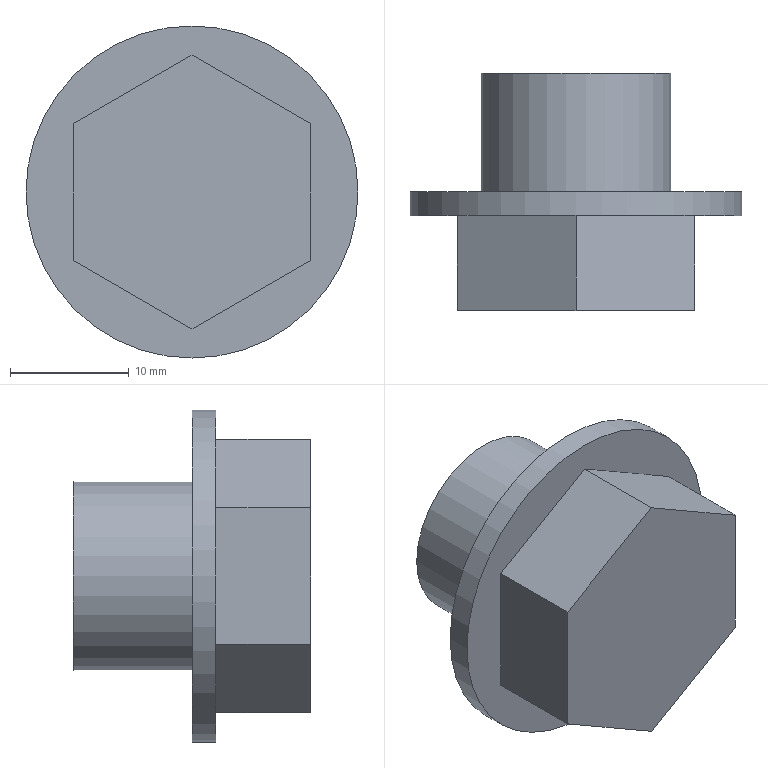Component | NX | LUOSAI | 1 solid | 12 faces | box 28 x 20 x 28 mm | volume 6013 mm3 | plane 10 | cylinder 2 | commonest cylinder face diameters 16 x1 28 x1
STEP:
#1=CARTESIAN_POINT('',(0.,0.,0.));
#2=DIRECTION('',(0.,0.,1.));
#3=DIRECTION('',(1.,0.,0.));
#4=AXIS2_PLACEMENT_3D('',#1,#2,#3);
#5=CARTESIAN_POINT('',(8.,-65.5,-196.));
#6=VERTEX_POINT('',#5);
#7=CARTESIAN_POINT('',(0.,-65.5,-196.));
#8=DIRECTION('',(0.,-1.,0.));
#9=DIRECTION('',(1.,0.,0.));
#10=AXIS2_PLACEMENT_3D('',#7,#8,#9);
#11=CIRCLE('',#10,8.);
#12=CARTESIAN_POINT('',(0.,-65.5,-196.));
#13=DIRECTION('',(0.,1.,0.));
#14=DIRECTION('',(0.,0.,1.));
#15=AXIS2_PLACEMENT_3D('',#12,#13,#14);
#16=CYLINDRICAL_SURFACE('',#15,8.);
#17=CARTESIAN_POINT('',(7.854,0.));
#18=DIRECTION('',(-1.,0.));
#19=VECTOR('',#18,1.);
#20=LINE('',#17,#19);
#21=(GEOMETRIC_REPRESENTATION_CONTEXT(2)PARAMETRIC_REPRESENTATION_CONTEXT()REPRESENTATION_CONTEXT('',''));
#22=DEFINITIONAL_REPRESENTATION('',(#20),#21);
#23=PCURVE('',#16,#22);
#24=CARTESIAN_POINT('',(0.,-65.5,-196.));
#25=DIRECTION('',(0.,-1.,0.));
#26=DIRECTION('',(0.,0.,-1.));
#27=AXIS2_PLACEMENT_3D('',#24,#25,#26);
#28=PLANE('',#27);
#29=CARTESIAN_POINT('',(0.,0.));
#30=DIRECTION('',(0.,1.));
#31=AXIS2_PLACEMENT_2D('',#29,#30);
#32=CIRCLE('',#31,8.);
#33=(GEOMETRIC_REPRESENTATION_CONTEXT(2)PARAMETRIC_REPRESENTATION_CONTEXT()REPRESENTATION_CONTEXT('',''));
#34=DEFINITIONAL_REPRESENTATION('',(#32),#33);
#35=PCURVE('',#28,#34);
#36=SURFACE_CURVE('',#11,(#23,#35),.PCURVE_S1.);
#37=EDGE_CURVE('',#6,#6,#36,.T.);
#38=ORIENTED_EDGE('',*,*,#37,.F.);
#39=CARTESIAN_POINT('',(8.,-55.5,-196.));
#40=VERTEX_POINT('',#39);
#41=CARTESIAN_POINT('',(8.,-65.5,-196.));
#42=CARTESIAN_POINT('',(8.,-55.5,-196.));
#43=B_SPLINE_CURVE_WITH_KNOTS('',1,(#41,#42),.UNSPECIFIED.,.F.,.F.,(2,2),(0.,10.),.PIECEWISE_BEZIER_KNOTS.);
#44=CARTESIAN_POINT('',(7.854,0.));
#45=DIRECTION('',(0.,1.));
#46=VECTOR('',#45,1.);
#47=LINE('',#44,#46);
#48=(GEOMETRIC_REPRESENTATION_CONTEXT(2)PARAMETRIC_REPRESENTATION_CONTEXT()REPRESENTATION_CONTEXT('',''));
#49=DEFINITIONAL_REPRESENTATION('',(#47),#48);
#50=PCURVE('',#16,#49);
#51=CARTESIAN_POINT('',(1.571,0.));
#52=DIRECTION('',(0.,1.));
#53=VECTOR('',#52,1.);
#54=LINE('',#51,#53);
#55=(GEOMETRIC_REPRESENTATION_CONTEXT(2)PARAMETRIC_REPRESENTATION_CONTEXT()REPRESENTATION_CONTEXT('',''));
#56=DEFINITIONAL_REPRESENTATION('',(#54),#55);
#57=PCURVE('',#16,#56);
#58=SEAM_CURVE('',#43,(#50,#57),.PCURVE_S1.);
#59=EDGE_CURVE('',#6,#40,#58,.T.);
#60=ORIENTED_EDGE('',*,*,#59,.T.);
#61=CARTESIAN_POINT('',(0.,-55.5,-196.));
#62=DIRECTION('',(0.,-1.,0.));
#63=DIRECTION('',(1.,0.,0.));
#64=AXIS2_PLACEMENT_3D('',#61,#62,#63);
#65=CIRCLE('',#64,8.);
#66=CARTESIAN_POINT('',(7.854,10.));
#67=DIRECTION('',(-1.,0.));
#68=VECTOR('',#67,1.);
#69=LINE('',#66,#68);
#70=(GEOMETRIC_REPRESENTATION_CONTEXT(2)PARAMETRIC_REPRESENTATION_CONTEXT()REPRESENTATION_CONTEXT('',''));
#71=DEFINITIONAL_REPRESENTATION('',(#69),#70);
#72=PCURVE('',#16,#71);
#73=CARTESIAN_POINT('',(0.,-55.5,-196.));
#74=DIRECTION('',(0.,-1.,0.));
#75=DIRECTION('',(0.,0.,-1.));
#76=AXIS2_PLACEMENT_3D('',#73,#74,#75);
#77=PLANE('',#76);
#78=CARTESIAN_POINT('',(0.,0.));
#79=DIRECTION('',(0.,1.));
#80=AXIS2_PLACEMENT_2D('',#78,#79);
#81=CIRCLE('',#80,8.);
#82=(GEOMETRIC_REPRESENTATION_CONTEXT(2)PARAMETRIC_REPRESENTATION_CONTEXT()REPRESENTATION_CONTEXT('',''));
#83=DEFINITIONAL_REPRESENTATION('',(#81),#82);
#84=PCURVE('',#77,#83);
#85=SURFACE_CURVE('',#65,(#72,#84),.PCURVE_S1.);
#86=EDGE_CURVE('',#40,#40,#85,.T.);
#87=ORIENTED_EDGE('',*,*,#86,.T.);
#88=ORIENTED_EDGE('',*,*,#59,.F.);
#89=EDGE_LOOP('',(#38,#60,#87,#88));
#90=FACE_BOUND('',#89,.T.);
#91=ADVANCED_FACE('',(#90),#16,.T.);
#92=ORIENTED_EDGE('',*,*,#86,.F.);
#93=EDGE_LOOP('',(#92));
#94=FACE_BOUND('',#93,.T.);
#95=ADVANCED_FACE('',(#94),#77,.F.);
#96=CARTESIAN_POINT('',(14.,-65.5,-196.));
#97=VERTEX_POINT('',#96);
#98=CARTESIAN_POINT('',(0.,-65.5,-196.));
#99=DIRECTION('',(0.,-1.,0.));
#100=DIRECTION('',(1.,0.,0.));
#101=AXIS2_PLACEMENT_3D('',#98,#99,#100);
#102=CIRCLE('',#101,14.);
#103=CARTESIAN_POINT('',(0.,0.));
#104=DIRECTION('',(0.,1.));
#105=AXIS2_PLACEMENT_2D('',#103,#104);
#106=CIRCLE('',#105,14.);
#107=(GEOMETRIC_REPRESENTATION_CONTEXT(2)PARAMETRIC_REPRESENTATION_CONTEXT()REPRESENTATION_CONTEXT('',''));
#108=DEFINITIONAL_REPRESENTATION('',(#106),#107);
#109=PCURVE('',#28,#108);
#110=CARTESIAN_POINT('',(0.,-67.5,-196.));
#111=DIRECTION('',(0.,1.,0.));
#112=DIRECTION('',(0.,0.,1.));
#113=AXIS2_PLACEMENT_3D('',#110,#111,#112);
#114=CYLINDRICAL_SURFACE('',#113,14.);
#115=CARTESIAN_POINT('',(7.854,2.));
#116=DIRECTION('',(-1.,0.));
#117=VECTOR('',#116,1.);
#118=LINE('',#115,#117);
#119=(GEOMETRIC_REPRESENTATION_CONTEXT(2)PARAMETRIC_REPRESENTATION_CONTEXT()REPRESENTATION_CONTEXT('',''));
#120=DEFINITIONAL_REPRESENTATION('',(#118),#119);
#121=PCURVE('',#114,#120);
#122=SURFACE_CURVE('',#102,(#109,#121),.PCURVE_S1.);
#123=EDGE_CURVE('',#97,#97,#122,.T.);
#124=ORIENTED_EDGE('',*,*,#123,.F.);
#125=EDGE_LOOP('',(#124));
#126=FACE_BOUND('',#125,.T.);
#127=ORIENTED_EDGE('',*,*,#37,.T.);
#128=EDGE_LOOP('',(#127));
#129=FACE_BOUND('',#128,.T.);
#130=ADVANCED_FACE('',(#126,#129),#28,.F.);
#131=CARTESIAN_POINT('',(14.,-67.5,-196.));
#132=VERTEX_POINT('',#131);
#133=CARTESIAN_POINT('',(0.,-67.5,-196.));
#134=DIRECTION('',(0.,-1.,0.));
#135=DIRECTION('',(1.,0.,0.));
#136=AXIS2_PLACEMENT_3D('',#133,#134,#135);
#137=CIRCLE('',#136,14.);
#138=CARTESIAN_POINT('',(7.854,0.));
#139=DIRECTION('',(-1.,0.));
#140=VECTOR('',#139,1.);
#141=LINE('',#138,#140);
#142=(GEOMETRIC_REPRESENTATION_CONTEXT(2)PARAMETRIC_REPRESENTATION_CONTEXT()REPRESENTATION_CONTEXT('',''));
#143=DEFINITIONAL_REPRESENTATION('',(#141),#142);
#144=PCURVE('',#114,#143);
#145=CARTESIAN_POINT('',(0.,-67.5,-196.));
#146=DIRECTION('',(0.,-1.,0.));
#147=DIRECTION('',(0.,0.,-1.));
#148=AXIS2_PLACEMENT_3D('',#145,#146,#147);
#149=PLANE('',#148);
#150=CARTESIAN_POINT('',(0.,0.));
#151=DIRECTION('',(0.,1.));
#152=AXIS2_PLACEMENT_2D('',#150,#151);
#153=CIRCLE('',#152,14.);
#154=(GEOMETRIC_REPRESENTATION_CONTEXT(2)PARAMETRIC_REPRESENTATION_CONTEXT()REPRESENTATION_CONTEXT('',''));
#155=DEFINITIONAL_REPRESENTATION('',(#153),#154);
#156=PCURVE('',#149,#155);
#157=SURFACE_CURVE('',#137,(#144,#156),.PCURVE_S1.);
#158=EDGE_CURVE('',#132,#132,#157,.T.);
#159=ORIENTED_EDGE('',*,*,#158,.F.);
#160=CARTESIAN_POINT('',(14.,-67.5,-196.));
#161=CARTESIAN_POINT('',(14.,-65.5,-196.));
#162=B_SPLINE_CURVE_WITH_KNOTS('',1,(#160,#161),.UNSPECIFIED.,.F.,.F.,(2,2),(0.,2.),.PIECEWISE_BEZIER_KNOTS.);
#163=CARTESIAN_POINT('',(7.854,0.));
#164=DIRECTION('',(0.,1.));
#165=VECTOR('',#164,1.);
#166=LINE('',#163,#165);
#167=(GEOMETRIC_REPRESENTATION_CONTEXT(2)PARAMETRIC_REPRESENTATION_CONTEXT()REPRESENTATION_CONTEXT('',''));
#168=DEFINITIONAL_REPRESENTATION('',(#166),#167);
#169=PCURVE('',#114,#168);
#170=CARTESIAN_POINT('',(1.571,0.));
#171=DIRECTION('',(0.,1.));
#172=VECTOR('',#171,1.);
#173=LINE('',#170,#172);
#174=(GEOMETRIC_REPRESENTATION_CONTEXT(2)PARAMETRIC_REPRESENTATION_CONTEXT()REPRESENTATION_CONTEXT('',''));
#175=DEFINITIONAL_REPRESENTATION('',(#173),#174);
#176=PCURVE('',#114,#175);
#177=SEAM_CURVE('',#162,(#169,#176),.PCURVE_S1.);
#178=EDGE_CURVE('',#132,#97,#177,.T.);
#179=ORIENTED_EDGE('',*,*,#178,.T.);
#180=ORIENTED_EDGE('',*,*,#123,.T.);
#181=ORIENTED_EDGE('',*,*,#178,.F.);
#182=EDGE_LOOP('',(#159,#179,#180,#181));
#183=FACE_BOUND('',#182,.T.);
#184=ADVANCED_FACE('',(#183),#114,.T.);
#185=CARTESIAN_POINT('',(-10.,-67.5,-190.226));
#186=VERTEX_POINT('',#185);
#187=CARTESIAN_POINT('',(-10.,-67.5,-201.774));
#188=VERTEX_POINT('',#187);
#189=CARTESIAN_POINT('',(-10.,-67.5,-190.226));
#190=DIRECTION('',(0.,0.,-1.));
#191=VECTOR('',#190,1.);
#192=LINE('',#189,#191);
#193=CARTESIAN_POINT('',(-5.774,-10.));
#194=DIRECTION('',(1.,0.));
#195=VECTOR('',#194,1.);
#196=LINE('',#193,#195);
#197=(GEOMETRIC_REPRESENTATION_CONTEXT(2)PARAMETRIC_REPRESENTATION_CONTEXT()REPRESENTATION_CONTEXT('',''));
#198=DEFINITIONAL_REPRESENTATION('',(#196),#197);
#199=PCURVE('',#149,#198);
#200=CARTESIAN_POINT('',(-10.,-75.5,-190.226));
#201=DIRECTION('',(1.,0.,0.));
#202=DIRECTION('',(0.,0.,1.));
#203=AXIS2_PLACEMENT_3D('',#200,#201,#202);
#204=PLANE('',#203);
#205=CARTESIAN_POINT('',(0.,-8.));
#206=DIRECTION('',(-1.,0.));
#207=VECTOR('',#206,1.);
#208=LINE('',#205,#207);
#209=(GEOMETRIC_REPRESENTATION_CONTEXT(2)PARAMETRIC_REPRESENTATION_CONTEXT()REPRESENTATION_CONTEXT('',''));
#210=DEFINITIONAL_REPRESENTATION('',(#208),#209);
#211=PCURVE('',#204,#210);
#212=SURFACE_CURVE('',#192,(#199,#211),.PCURVE_S1.);
#213=EDGE_CURVE('',#186,#188,#212,.T.);
#214=ORIENTED_EDGE('',*,*,#213,.F.);
#215=CARTESIAN_POINT('',(0.,-67.5,-184.453));
#216=VERTEX_POINT('',#215);
#217=CARTESIAN_POINT('',(0.,-67.5,-184.453));
#218=DIRECTION('',(-0.866,0.,-0.5));
#219=VECTOR('',#218,1.);
#220=LINE('',#217,#219);
#221=CARTESIAN_POINT('',(-11.547,0.));
#222=DIRECTION('',(0.5,-0.866));
#223=VECTOR('',#222,1.);
#224=LINE('',#221,#223);
#225=(GEOMETRIC_REPRESENTATION_CONTEXT(2)PARAMETRIC_REPRESENTATION_CONTEXT()REPRESENTATION_CONTEXT('',''));
#226=DEFINITIONAL_REPRESENTATION('',(#224),#225);
#227=PCURVE('',#149,#226);
#228=CARTESIAN_POINT('',(0.,-75.5,-184.453));
#229=DIRECTION('',(0.5,0.,-0.866));
#230=DIRECTION('',(0.866,0.,0.5));
#231=AXIS2_PLACEMENT_3D('',#228,#229,#230);
#232=PLANE('',#231);
#233=CARTESIAN_POINT('',(0.,-8.));
#234=DIRECTION('',(-1.,0.));
#235=VECTOR('',#234,1.);
#236=LINE('',#233,#235);
#237=(GEOMETRIC_REPRESENTATION_CONTEXT(2)PARAMETRIC_REPRESENTATION_CONTEXT()REPRESENTATION_CONTEXT('',''));
#238=DEFINITIONAL_REPRESENTATION('',(#236),#237);
#239=PCURVE('',#232,#238);
#240=SURFACE_CURVE('',#220,(#227,#239),.PCURVE_S1.);
#241=EDGE_CURVE('',#216,#186,#240,.T.);
#242=ORIENTED_EDGE('',*,*,#241,.F.);
#243=CARTESIAN_POINT('',(10.,-67.5,-190.226));
#244=VERTEX_POINT('',#243);
#245=CARTESIAN_POINT('',(10.,-67.5,-190.226));
#246=DIRECTION('',(-0.866,0.,0.5));
#247=VECTOR('',#246,1.);
#248=LINE('',#245,#247);
#249=CARTESIAN_POINT('',(-5.774,10.));
#250=DIRECTION('',(-0.5,-0.866));
#251=VECTOR('',#250,1.);
#252=LINE('',#249,#251);
#253=(GEOMETRIC_REPRESENTATION_CONTEXT(2)PARAMETRIC_REPRESENTATION_CONTEXT()REPRESENTATION_CONTEXT('',''));
#254=DEFINITIONAL_REPRESENTATION('',(#252),#253);
#255=PCURVE('',#149,#254);
#256=CARTESIAN_POINT('',(10.,-75.5,-190.226));
#257=DIRECTION('',(-0.5,0.,-0.866));
#258=DIRECTION('',(0.866,0.,-0.5));
#259=AXIS2_PLACEMENT_3D('',#256,#257,#258);
#260=PLANE('',#259);
#261=CARTESIAN_POINT('',(0.,-8.));
#262=DIRECTION('',(-1.,0.));
#263=VECTOR('',#262,1.);
#264=LINE('',#261,#263);
#265=(GEOMETRIC_REPRESENTATION_CONTEXT(2)PARAMETRIC_REPRESENTATION_CONTEXT()REPRESENTATION_CONTEXT('',''));
#266=DEFINITIONAL_REPRESENTATION('',(#264),#265);
#267=PCURVE('',#260,#266);
#268=SURFACE_CURVE('',#248,(#255,#267),.PCURVE_S1.);
#269=EDGE_CURVE('',#244,#216,#268,.T.);
#270=ORIENTED_EDGE('',*,*,#269,.F.);
#271=CARTESIAN_POINT('',(10.,-67.5,-201.774));
#272=VERTEX_POINT('',#271);
#273=CARTESIAN_POINT('',(10.,-67.5,-201.774));
#274=DIRECTION('',(0.,0.,1.));
#275=VECTOR('',#274,1.);
#276=LINE('',#273,#275);
#277=CARTESIAN_POINT('',(5.774,10.));
#278=DIRECTION('',(-1.,0.));
#279=VECTOR('',#278,1.);
#280=LINE('',#277,#279);
#281=(GEOMETRIC_REPRESENTATION_CONTEXT(2)PARAMETRIC_REPRESENTATION_CONTEXT()REPRESENTATION_CONTEXT('',''));
#282=DEFINITIONAL_REPRESENTATION('',(#280),#281);
#283=PCURVE('',#149,#282);
#284=CARTESIAN_POINT('',(10.,-75.5,-201.774));
#285=DIRECTION('',(-1.,0.,0.));
#286=DIRECTION('',(0.,0.,-1.));
#287=AXIS2_PLACEMENT_3D('',#284,#285,#286);
#288=PLANE('',#287);
#289=CARTESIAN_POINT('',(0.,-8.));
#290=DIRECTION('',(-1.,0.));
#291=VECTOR('',#290,1.);
#292=LINE('',#289,#291);
#293=(GEOMETRIC_REPRESENTATION_CONTEXT(2)PARAMETRIC_REPRESENTATION_CONTEXT()REPRESENTATION_CONTEXT('',''));
#294=DEFINITIONAL_REPRESENTATION('',(#292),#293);
#295=PCURVE('',#288,#294);
#296=SURFACE_CURVE('',#276,(#283,#295),.PCURVE_S1.);
#297=EDGE_CURVE('',#272,#244,#296,.T.);
#298=ORIENTED_EDGE('',*,*,#297,.F.);
#299=CARTESIAN_POINT('',(-0.,-67.5,-207.547));
#300=VERTEX_POINT('',#299);
#301=CARTESIAN_POINT('',(-0.,-67.5,-207.547));
#302=DIRECTION('',(0.866,0.,0.5));
#303=VECTOR('',#302,1.);
#304=LINE('',#301,#303);
#305=CARTESIAN_POINT('',(11.547,-0.));
#306=DIRECTION('',(-0.5,0.866));
#307=VECTOR('',#306,1.);
#308=LINE('',#305,#307);
#309=(GEOMETRIC_REPRESENTATION_CONTEXT(2)PARAMETRIC_REPRESENTATION_CONTEXT()REPRESENTATION_CONTEXT('',''));
#310=DEFINITIONAL_REPRESENTATION('',(#308),#309);
#311=PCURVE('',#149,#310);
#312=CARTESIAN_POINT('',(-0.,-75.5,-207.547));
#313=DIRECTION('',(-0.5,0.,0.866));
#314=DIRECTION('',(-0.866,0.,-0.5));
#315=AXIS2_PLACEMENT_3D('',#312,#313,#314);
#316=PLANE('',#315);
#317=CARTESIAN_POINT('',(0.,-8.));
#318=DIRECTION('',(-1.,0.));
#319=VECTOR('',#318,1.);
#320=LINE('',#317,#319);
#321=(GEOMETRIC_REPRESENTATION_CONTEXT(2)PARAMETRIC_REPRESENTATION_CONTEXT()REPRESENTATION_CONTEXT('',''));
#322=DEFINITIONAL_REPRESENTATION('',(#320),#321);
#323=PCURVE('',#316,#322);
#324=SURFACE_CURVE('',#304,(#311,#323),.PCURVE_S1.);
#325=EDGE_CURVE('',#300,#272,#324,.T.);
#326=ORIENTED_EDGE('',*,*,#325,.F.);
#327=CARTESIAN_POINT('',(-10.,-67.5,-201.774));
#328=DIRECTION('',(0.866,0.,-0.5));
#329=VECTOR('',#328,1.);
#330=LINE('',#327,#329);
#331=CARTESIAN_POINT('',(5.774,-10.));
#332=DIRECTION('',(0.5,0.866));
#333=VECTOR('',#332,1.);
#334=LINE('',#331,#333);
#335=(GEOMETRIC_REPRESENTATION_CONTEXT(2)PARAMETRIC_REPRESENTATION_CONTEXT()REPRESENTATION_CONTEXT('',''));
#336=DEFINITIONAL_REPRESENTATION('',(#334),#335);
#337=PCURVE('',#149,#336);
#338=CARTESIAN_POINT('',(-10.,-75.5,-201.774));
#339=DIRECTION('',(0.5,0.,0.866));
#340=DIRECTION('',(-0.866,0.,0.5));
#341=AXIS2_PLACEMENT_3D('',#338,#339,#340);
#342=PLANE('',#341);
#343=CARTESIAN_POINT('',(0.,-8.));
#344=DIRECTION('',(-1.,0.));
#345=VECTOR('',#344,1.);
#346=LINE('',#343,#345);
#347=(GEOMETRIC_REPRESENTATION_CONTEXT(2)PARAMETRIC_REPRESENTATION_CONTEXT()REPRESENTATION_CONTEXT('',''));
#348=DEFINITIONAL_REPRESENTATION('',(#346),#347);
#349=PCURVE('',#342,#348);
#350=SURFACE_CURVE('',#330,(#337,#349),.PCURVE_S1.);
#351=EDGE_CURVE('',#188,#300,#350,.T.);
#352=ORIENTED_EDGE('',*,*,#351,.F.);
#353=EDGE_LOOP('',(#214,#242,#270,#298,#326,#352));
#354=FACE_BOUND('',#353,.T.);
#355=ORIENTED_EDGE('',*,*,#158,.T.);
#356=EDGE_LOOP('',(#355));
#357=FACE_BOUND('',#356,.T.);
#358=ADVANCED_FACE('',(#354,#357),#149,.T.);
#359=ORIENTED_EDGE('',*,*,#213,.T.);
#360=CARTESIAN_POINT('',(-10.,-75.5,-201.774));
#361=VERTEX_POINT('',#360);
#362=CARTESIAN_POINT('',(-10.,-75.5,-201.774));
#363=DIRECTION('',(0.,1.,0.));
#364=VECTOR('',#363,1.);
#365=LINE('',#362,#364);
#366=CARTESIAN_POINT('',(-11.547,0.));
#367=DIRECTION('',(0.,-1.));
#368=VECTOR('',#367,1.);
#369=LINE('',#366,#368);
#370=(GEOMETRIC_REPRESENTATION_CONTEXT(2)PARAMETRIC_REPRESENTATION_CONTEXT()REPRESENTATION_CONTEXT('',''));
#371=DEFINITIONAL_REPRESENTATION('',(#369),#370);
#372=PCURVE('',#204,#371);
#373=CARTESIAN_POINT('',(-0.,0.));
#374=DIRECTION('',(0.,-1.));
#375=VECTOR('',#374,1.);
#376=LINE('',#373,#375);
#377=(GEOMETRIC_REPRESENTATION_CONTEXT(2)PARAMETRIC_REPRESENTATION_CONTEXT()REPRESENTATION_CONTEXT('',''));
#378=DEFINITIONAL_REPRESENTATION('',(#376),#377);
#379=PCURVE('',#342,#378);
#380=SURFACE_CURVE('',#365,(#372,#379),.PCURVE_S1.);
#381=EDGE_CURVE('',#361,#188,#380,.T.);
#382=ORIENTED_EDGE('',*,*,#381,.F.);
#383=CARTESIAN_POINT('',(-10.,-75.5,-190.226));
#384=VERTEX_POINT('',#383);
#385=CARTESIAN_POINT('',(-10.,-75.5,-190.226));
#386=DIRECTION('',(0.,0.,-1.));
#387=VECTOR('',#386,1.);
#388=LINE('',#385,#387);
#389=CARTESIAN_POINT('',(0.,0.));
#390=DIRECTION('',(-1.,0.));
#391=VECTOR('',#390,1.);
#392=LINE('',#389,#391);
#393=(GEOMETRIC_REPRESENTATION_CONTEXT(2)PARAMETRIC_REPRESENTATION_CONTEXT()REPRESENTATION_CONTEXT('',''));
#394=DEFINITIONAL_REPRESENTATION('',(#392),#393);
#395=PCURVE('',#204,#394);
#396=CARTESIAN_POINT('',(0.,-75.5,-196.));
#397=DIRECTION('',(0.,-1.,0.));
#398=DIRECTION('',(0.,0.,-1.));
#399=AXIS2_PLACEMENT_3D('',#396,#397,#398);
#400=PLANE('',#399);
#401=CARTESIAN_POINT('',(-5.774,-10.));
#402=DIRECTION('',(1.,0.));
#403=VECTOR('',#402,1.);
#404=LINE('',#401,#403);
#405=(GEOMETRIC_REPRESENTATION_CONTEXT(2)PARAMETRIC_REPRESENTATION_CONTEXT()REPRESENTATION_CONTEXT('',''));
#406=DEFINITIONAL_REPRESENTATION('',(#404),#405);
#407=PCURVE('',#400,#406);
#408=SURFACE_CURVE('',#388,(#395,#407),.PCURVE_S1.);
#409=EDGE_CURVE('',#384,#361,#408,.T.);
#410=ORIENTED_EDGE('',*,*,#409,.F.);
#411=CARTESIAN_POINT('',(-10.,-75.5,-190.226));
#412=DIRECTION('',(0.,1.,0.));
#413=VECTOR('',#412,1.);
#414=LINE('',#411,#413);
#415=CARTESIAN_POINT('',(0.,0.));
#416=DIRECTION('',(0.,-1.));
#417=VECTOR('',#416,1.);
#418=LINE('',#415,#417);
#419=(GEOMETRIC_REPRESENTATION_CONTEXT(2)PARAMETRIC_REPRESENTATION_CONTEXT()REPRESENTATION_CONTEXT('',''));
#420=DEFINITIONAL_REPRESENTATION('',(#418),#419);
#421=PCURVE('',#204,#420);
#422=CARTESIAN_POINT('',(-11.547,0.));
#423=DIRECTION('',(0.,-1.));
#424=VECTOR('',#423,1.);
#425=LINE('',#422,#424);
#426=(GEOMETRIC_REPRESENTATION_CONTEXT(2)PARAMETRIC_REPRESENTATION_CONTEXT()REPRESENTATION_CONTEXT('',''));
#427=DEFINITIONAL_REPRESENTATION('',(#425),#426);
#428=PCURVE('',#232,#427);
#429=SURFACE_CURVE('',#414,(#421,#428),.PCURVE_S1.);
#430=EDGE_CURVE('',#384,#186,#429,.T.);
#431=ORIENTED_EDGE('',*,*,#430,.T.);
#432=EDGE_LOOP('',(#359,#382,#410,#431));
#433=FACE_BOUND('',#432,.T.);
#434=ADVANCED_FACE('',(#433),#204,.F.);
#435=ORIENTED_EDGE('',*,*,#351,.T.);
#436=CARTESIAN_POINT('',(-0.,-75.5,-207.547));
#437=VERTEX_POINT('',#436);
#438=CARTESIAN_POINT('',(-0.,-75.5,-207.547));
#439=DIRECTION('',(0.,1.,0.));
#440=VECTOR('',#439,1.);
#441=LINE('',#438,#440);
#442=CARTESIAN_POINT('',(-11.547,0.));
#443=DIRECTION('',(0.,-1.));
#444=VECTOR('',#443,1.);
#445=LINE('',#442,#444);
#446=(GEOMETRIC_REPRESENTATION_CONTEXT(2)PARAMETRIC_REPRESENTATION_CONTEXT()REPRESENTATION_CONTEXT('',''));
#447=DEFINITIONAL_REPRESENTATION('',(#445),#446);
#448=PCURVE('',#342,#447);
#449=CARTESIAN_POINT('',(-0.,0.));
#450=DIRECTION('',(0.,-1.));
#451=VECTOR('',#450,1.);
#452=LINE('',#449,#451);
#453=(GEOMETRIC_REPRESENTATION_CONTEXT(2)PARAMETRIC_REPRESENTATION_CONTEXT()REPRESENTATION_CONTEXT('',''));
#454=DEFINITIONAL_REPRESENTATION('',(#452),#453);
#455=PCURVE('',#316,#454);
#456=SURFACE_CURVE('',#441,(#448,#455),.PCURVE_S1.);
#457=EDGE_CURVE('',#437,#300,#456,.T.);
#458=ORIENTED_EDGE('',*,*,#457,.F.);
#459=CARTESIAN_POINT('',(-10.,-75.5,-201.774));
#460=DIRECTION('',(0.866,0.,-0.5));
#461=VECTOR('',#460,1.);
#462=LINE('',#459,#461);
#463=CARTESIAN_POINT('',(0.,0.));
#464=DIRECTION('',(-1.,0.));
#465=VECTOR('',#464,1.);
#466=LINE('',#463,#465);
#467=(GEOMETRIC_REPRESENTATION_CONTEXT(2)PARAMETRIC_REPRESENTATION_CONTEXT()REPRESENTATION_CONTEXT('',''));
#468=DEFINITIONAL_REPRESENTATION('',(#466),#467);
#469=PCURVE('',#342,#468);
#470=CARTESIAN_POINT('',(5.774,-10.));
#471=DIRECTION('',(0.5,0.866));
#472=VECTOR('',#471,1.);
#473=LINE('',#470,#472);
#474=(GEOMETRIC_REPRESENTATION_CONTEXT(2)PARAMETRIC_REPRESENTATION_CONTEXT()REPRESENTATION_CONTEXT('',''));
#475=DEFINITIONAL_REPRESENTATION('',(#473),#474);
#476=PCURVE('',#400,#475);
#477=SURFACE_CURVE('',#462,(#469,#476),.PCURVE_S1.);
#478=EDGE_CURVE('',#361,#437,#477,.T.);
#479=ORIENTED_EDGE('',*,*,#478,.F.);
#480=ORIENTED_EDGE('',*,*,#381,.T.);
#481=EDGE_LOOP('',(#435,#458,#479,#480));
#482=FACE_BOUND('',#481,.T.);
#483=ADVANCED_FACE('',(#482),#342,.F.);
#484=ORIENTED_EDGE('',*,*,#325,.T.);
#485=CARTESIAN_POINT('',(10.,-75.5,-201.774));
#486=VERTEX_POINT('',#485);
#487=CARTESIAN_POINT('',(10.,-75.5,-201.774));
#488=DIRECTION('',(0.,1.,0.));
#489=VECTOR('',#488,1.);
#490=LINE('',#487,#489);
#491=CARTESIAN_POINT('',(-11.547,0.));
#492=DIRECTION('',(0.,-1.));
#493=VECTOR('',#492,1.);
#494=LINE('',#491,#493);
#495=(GEOMETRIC_REPRESENTATION_CONTEXT(2)PARAMETRIC_REPRESENTATION_CONTEXT()REPRESENTATION_CONTEXT('',''));
#496=DEFINITIONAL_REPRESENTATION('',(#494),#495);
#497=PCURVE('',#316,#496);
#498=CARTESIAN_POINT('',(0.,0.));
#499=DIRECTION('',(0.,-1.));
#500=VECTOR('',#499,1.);
#501=LINE('',#498,#500);
#502=(GEOMETRIC_REPRESENTATION_CONTEXT(2)PARAMETRIC_REPRESENTATION_CONTEXT()REPRESENTATION_CONTEXT('',''));
#503=DEFINITIONAL_REPRESENTATION('',(#501),#502);
#504=PCURVE('',#288,#503);
#505=SURFACE_CURVE('',#490,(#497,#504),.PCURVE_S1.);
#506=EDGE_CURVE('',#486,#272,#505,.T.);
#507=ORIENTED_EDGE('',*,*,#506,.F.);
#508=CARTESIAN_POINT('',(-0.,-75.5,-207.547));
#509=DIRECTION('',(0.866,0.,0.5));
#510=VECTOR('',#509,1.);
#511=LINE('',#508,#510);
#512=CARTESIAN_POINT('',(0.,0.));
#513=DIRECTION('',(-1.,0.));
#514=VECTOR('',#513,1.);
#515=LINE('',#512,#514);
#516=(GEOMETRIC_REPRESENTATION_CONTEXT(2)PARAMETRIC_REPRESENTATION_CONTEXT()REPRESENTATION_CONTEXT('',''));
#517=DEFINITIONAL_REPRESENTATION('',(#515),#516);
#518=PCURVE('',#316,#517);
#519=CARTESIAN_POINT('',(11.547,-0.));
#520=DIRECTION('',(-0.5,0.866));
#521=VECTOR('',#520,1.);
#522=LINE('',#519,#521);
#523=(GEOMETRIC_REPRESENTATION_CONTEXT(2)PARAMETRIC_REPRESENTATION_CONTEXT()REPRESENTATION_CONTEXT('',''));
#524=DEFINITIONAL_REPRESENTATION('',(#522),#523);
#525=PCURVE('',#400,#524);
#526=SURFACE_CURVE('',#511,(#518,#525),.PCURVE_S1.);
#527=EDGE_CURVE('',#437,#486,#526,.T.);
#528=ORIENTED_EDGE('',*,*,#527,.F.);
#529=ORIENTED_EDGE('',*,*,#457,.T.);
#530=EDGE_LOOP('',(#484,#507,#528,#529));
#531=FACE_BOUND('',#530,.T.);
#532=ADVANCED_FACE('',(#531),#316,.F.);
#533=ORIENTED_EDGE('',*,*,#297,.T.);
#534=CARTESIAN_POINT('',(10.,-75.5,-190.226));
#535=VERTEX_POINT('',#534);
#536=CARTESIAN_POINT('',(10.,-75.5,-190.226));
#537=DIRECTION('',(0.,1.,0.));
#538=VECTOR('',#537,1.);
#539=LINE('',#536,#538);
#540=CARTESIAN_POINT('',(-11.547,0.));
#541=DIRECTION('',(0.,-1.));
#542=VECTOR('',#541,1.);
#543=LINE('',#540,#542);
#544=(GEOMETRIC_REPRESENTATION_CONTEXT(2)PARAMETRIC_REPRESENTATION_CONTEXT()REPRESENTATION_CONTEXT('',''));
#545=DEFINITIONAL_REPRESENTATION('',(#543),#544);
#546=PCURVE('',#288,#545);
#547=CARTESIAN_POINT('',(0.,0.));
#548=DIRECTION('',(0.,-1.));
#549=VECTOR('',#548,1.);
#550=LINE('',#547,#549);
#551=(GEOMETRIC_REPRESENTATION_CONTEXT(2)PARAMETRIC_REPRESENTATION_CONTEXT()REPRESENTATION_CONTEXT('',''));
#552=DEFINITIONAL_REPRESENTATION('',(#550),#551);
#553=PCURVE('',#260,#552);
#554=SURFACE_CURVE('',#539,(#546,#553),.PCURVE_S1.);
#555=EDGE_CURVE('',#535,#244,#554,.T.);
#556=ORIENTED_EDGE('',*,*,#555,.F.);
#557=CARTESIAN_POINT('',(10.,-75.5,-201.774));
#558=DIRECTION('',(0.,0.,1.));
#559=VECTOR('',#558,1.);
#560=LINE('',#557,#559);
#561=CARTESIAN_POINT('',(0.,0.));
#562=DIRECTION('',(-1.,0.));
#563=VECTOR('',#562,1.);
#564=LINE('',#561,#563);
#565=(GEOMETRIC_REPRESENTATION_CONTEXT(2)PARAMETRIC_REPRESENTATION_CONTEXT()REPRESENTATION_CONTEXT('',''));
#566=DEFINITIONAL_REPRESENTATION('',(#564),#565);
#567=PCURVE('',#288,#566);
#568=CARTESIAN_POINT('',(5.774,10.));
#569=DIRECTION('',(-1.,0.));
#570=VECTOR('',#569,1.);
#571=LINE('',#568,#570);
#572=(GEOMETRIC_REPRESENTATION_CONTEXT(2)PARAMETRIC_REPRESENTATION_CONTEXT()REPRESENTATION_CONTEXT('',''));
#573=DEFINITIONAL_REPRESENTATION('',(#571),#572);
#574=PCURVE('',#400,#573);
#575=SURFACE_CURVE('',#560,(#567,#574),.PCURVE_S1.);
#576=EDGE_CURVE('',#486,#535,#575,.T.);
#577=ORIENTED_EDGE('',*,*,#576,.F.);
#578=ORIENTED_EDGE('',*,*,#506,.T.);
#579=EDGE_LOOP('',(#533,#556,#577,#578));
#580=FACE_BOUND('',#579,.T.);
#581=ADVANCED_FACE('',(#580),#288,.F.);
#582=ORIENTED_EDGE('',*,*,#269,.T.);
#583=CARTESIAN_POINT('',(0.,-75.5,-184.453));
#584=VERTEX_POINT('',#583);
#585=CARTESIAN_POINT('',(0.,-75.5,-184.453));
#586=DIRECTION('',(0.,1.,0.));
#587=VECTOR('',#586,1.);
#588=LINE('',#585,#587);
#589=CARTESIAN_POINT('',(-11.547,0.));
#590=DIRECTION('',(0.,-1.));
#591=VECTOR('',#590,1.);
#592=LINE('',#589,#591);
#593=(GEOMETRIC_REPRESENTATION_CONTEXT(2)PARAMETRIC_REPRESENTATION_CONTEXT()REPRESENTATION_CONTEXT('',''));
#594=DEFINITIONAL_REPRESENTATION('',(#592),#593);
#595=PCURVE('',#260,#594);
#596=CARTESIAN_POINT('',(0.,0.));
#597=DIRECTION('',(0.,-1.));
#598=VECTOR('',#597,1.);
#599=LINE('',#596,#598);
#600=(GEOMETRIC_REPRESENTATION_CONTEXT(2)PARAMETRIC_REPRESENTATION_CONTEXT()REPRESENTATION_CONTEXT('',''));
#601=DEFINITIONAL_REPRESENTATION('',(#599),#600);
#602=PCURVE('',#232,#601);
#603=SURFACE_CURVE('',#588,(#595,#602),.PCURVE_S1.);
#604=EDGE_CURVE('',#584,#216,#603,.T.);
#605=ORIENTED_EDGE('',*,*,#604,.F.);
#606=CARTESIAN_POINT('',(10.,-75.5,-190.226));
#607=DIRECTION('',(-0.866,0.,0.5));
#608=VECTOR('',#607,1.);
#609=LINE('',#606,#608);
#610=CARTESIAN_POINT('',(0.,0.));
#611=DIRECTION('',(-1.,0.));
#612=VECTOR('',#611,1.);
#613=LINE('',#610,#612);
#614=(GEOMETRIC_REPRESENTATION_CONTEXT(2)PARAMETRIC_REPRESENTATION_CONTEXT()REPRESENTATION_CONTEXT('',''));
#615=DEFINITIONAL_REPRESENTATION('',(#613),#614);
#616=PCURVE('',#260,#615);
#617=CARTESIAN_POINT('',(-5.774,10.));
#618=DIRECTION('',(-0.5,-0.866));
#619=VECTOR('',#618,1.);
#620=LINE('',#617,#619);
#621=(GEOMETRIC_REPRESENTATION_CONTEXT(2)PARAMETRIC_REPRESENTATION_CONTEXT()REPRESENTATION_CONTEXT('',''));
#622=DEFINITIONAL_REPRESENTATION('',(#620),#621);
#623=PCURVE('',#400,#622);
#624=SURFACE_CURVE('',#609,(#616,#623),.PCURVE_S1.);
#625=EDGE_CURVE('',#535,#584,#624,.T.);
#626=ORIENTED_EDGE('',*,*,#625,.F.);
#627=ORIENTED_EDGE('',*,*,#555,.T.);
#628=EDGE_LOOP('',(#582,#605,#626,#627));
#629=FACE_BOUND('',#628,.T.);
#630=ADVANCED_FACE('',(#629),#260,.F.);
#631=ORIENTED_EDGE('',*,*,#241,.T.);
#632=ORIENTED_EDGE('',*,*,#430,.F.);
#633=CARTESIAN_POINT('',(0.,-75.5,-184.453));
#634=DIRECTION('',(-0.866,0.,-0.5));
#635=VECTOR('',#634,1.);
#636=LINE('',#633,#635);
#637=CARTESIAN_POINT('',(0.,0.));
#638=DIRECTION('',(-1.,0.));
#639=VECTOR('',#638,1.);
#640=LINE('',#637,#639);
#641=(GEOMETRIC_REPRESENTATION_CONTEXT(2)PARAMETRIC_REPRESENTATION_CONTEXT()REPRESENTATION_CONTEXT('',''));
#642=DEFINITIONAL_REPRESENTATION('',(#640),#641);
#643=PCURVE('',#232,#642);
#644=CARTESIAN_POINT('',(-11.547,0.));
#645=DIRECTION('',(0.5,-0.866));
#646=VECTOR('',#645,1.);
#647=LINE('',#644,#646);
#648=(GEOMETRIC_REPRESENTATION_CONTEXT(2)PARAMETRIC_REPRESENTATION_CONTEXT()REPRESENTATION_CONTEXT('',''));
#649=DEFINITIONAL_REPRESENTATION('',(#647),#648);
#650=PCURVE('',#400,#649);
#651=SURFACE_CURVE('',#636,(#643,#650),.PCURVE_S1.);
#652=EDGE_CURVE('',#584,#384,#651,.T.);
#653=ORIENTED_EDGE('',*,*,#652,.F.);
#654=ORIENTED_EDGE('',*,*,#604,.T.);
#655=EDGE_LOOP('',(#631,#632,#653,#654));
#656=FACE_BOUND('',#655,.T.);
#657=ADVANCED_FACE('',(#656),#232,.F.);
#658=ORIENTED_EDGE('',*,*,#409,.T.);
#659=ORIENTED_EDGE('',*,*,#478,.T.);
#660=ORIENTED_EDGE('',*,*,#527,.T.);
#661=ORIENTED_EDGE('',*,*,#576,.T.);
#662=ORIENTED_EDGE('',*,*,#625,.T.);
#663=ORIENTED_EDGE('',*,*,#652,.T.);
#664=EDGE_LOOP('',(#658,#659,#660,#661,#662,#663));
#665=FACE_BOUND('',#664,.T.);
#666=ADVANCED_FACE('',(#665),#400,.T.);
#667=CLOSED_SHELL('',(#91,#95,#130,#184,#358,#434,#483,#532,#581,#630,#657,#666));
#668=MANIFOLD_SOLID_BREP('',#667);
#669=(LENGTH_UNIT()NAMED_UNIT(*)SI_UNIT(.MILLI.,.METRE.));
#670=UNCERTAINTY_MEASURE_WITH_UNIT(LENGTH_MEASURE(0.000002),#669,'','');
#671=(NAMED_UNIT(*)PLANE_ANGLE_UNIT()SI_UNIT($,.RADIAN.));
#672=(NAMED_UNIT(*)SI_UNIT($,.STERADIAN.)SOLID_ANGLE_UNIT());
#673=(GEOMETRIC_REPRESENTATION_CONTEXT(3)GLOBAL_UNCERTAINTY_ASSIGNED_CONTEXT((#670))GLOBAL_UNIT_ASSIGNED_CONTEXT((#669,#671,#672))REPRESENTATION_CONTEXT('',''));
#674=ADVANCED_BREP_SHAPE_REPRESENTATION('',(#4,#668),#673);